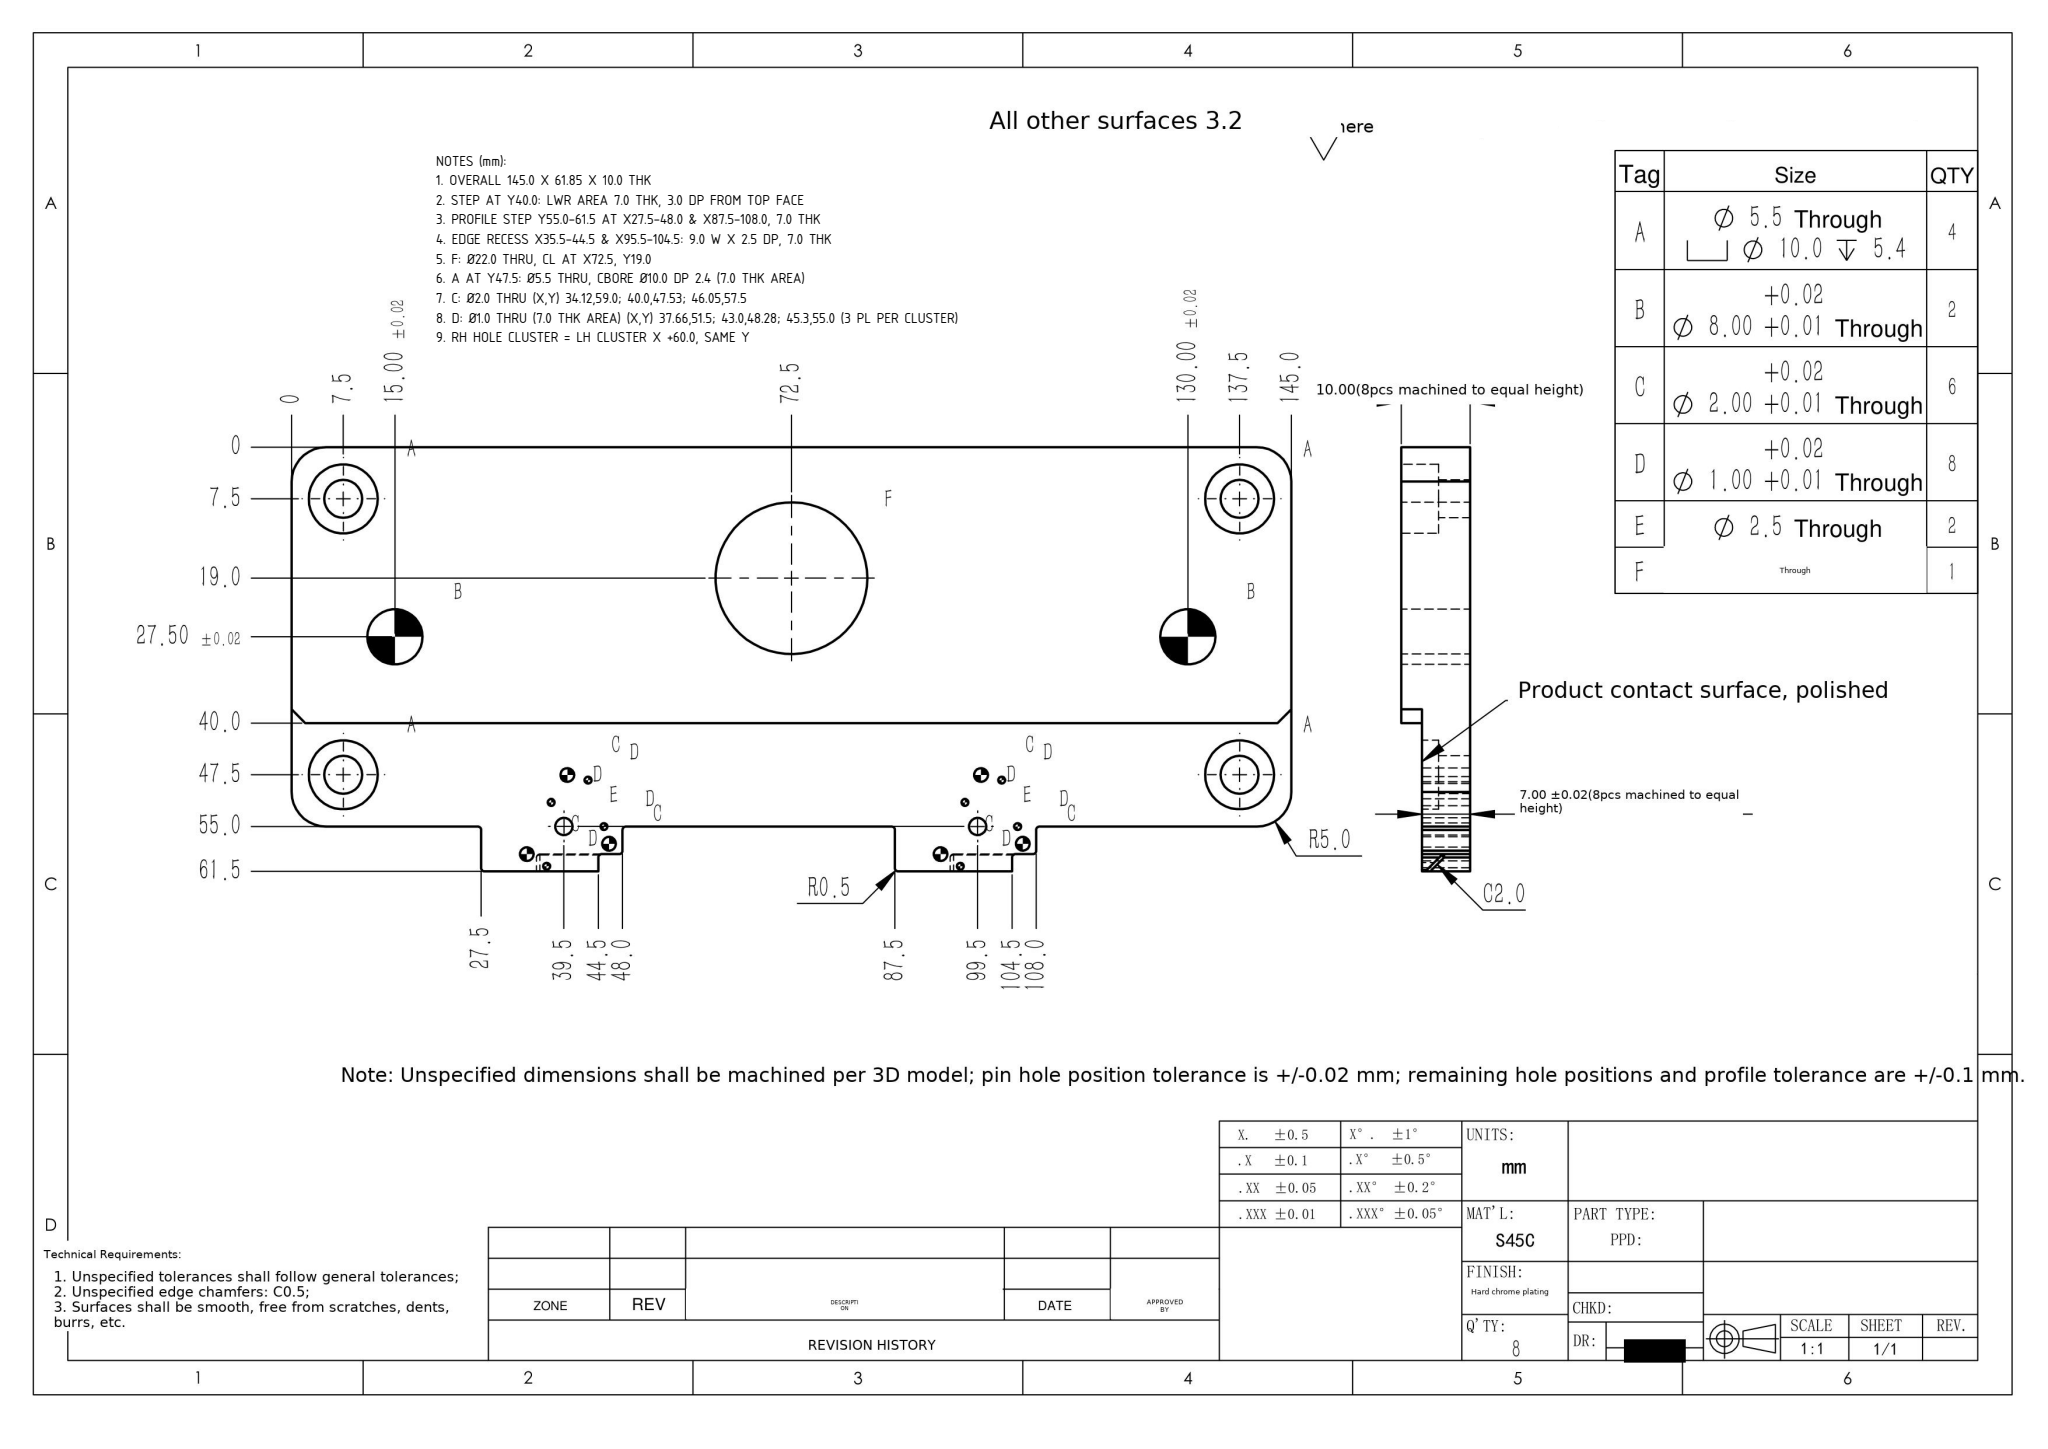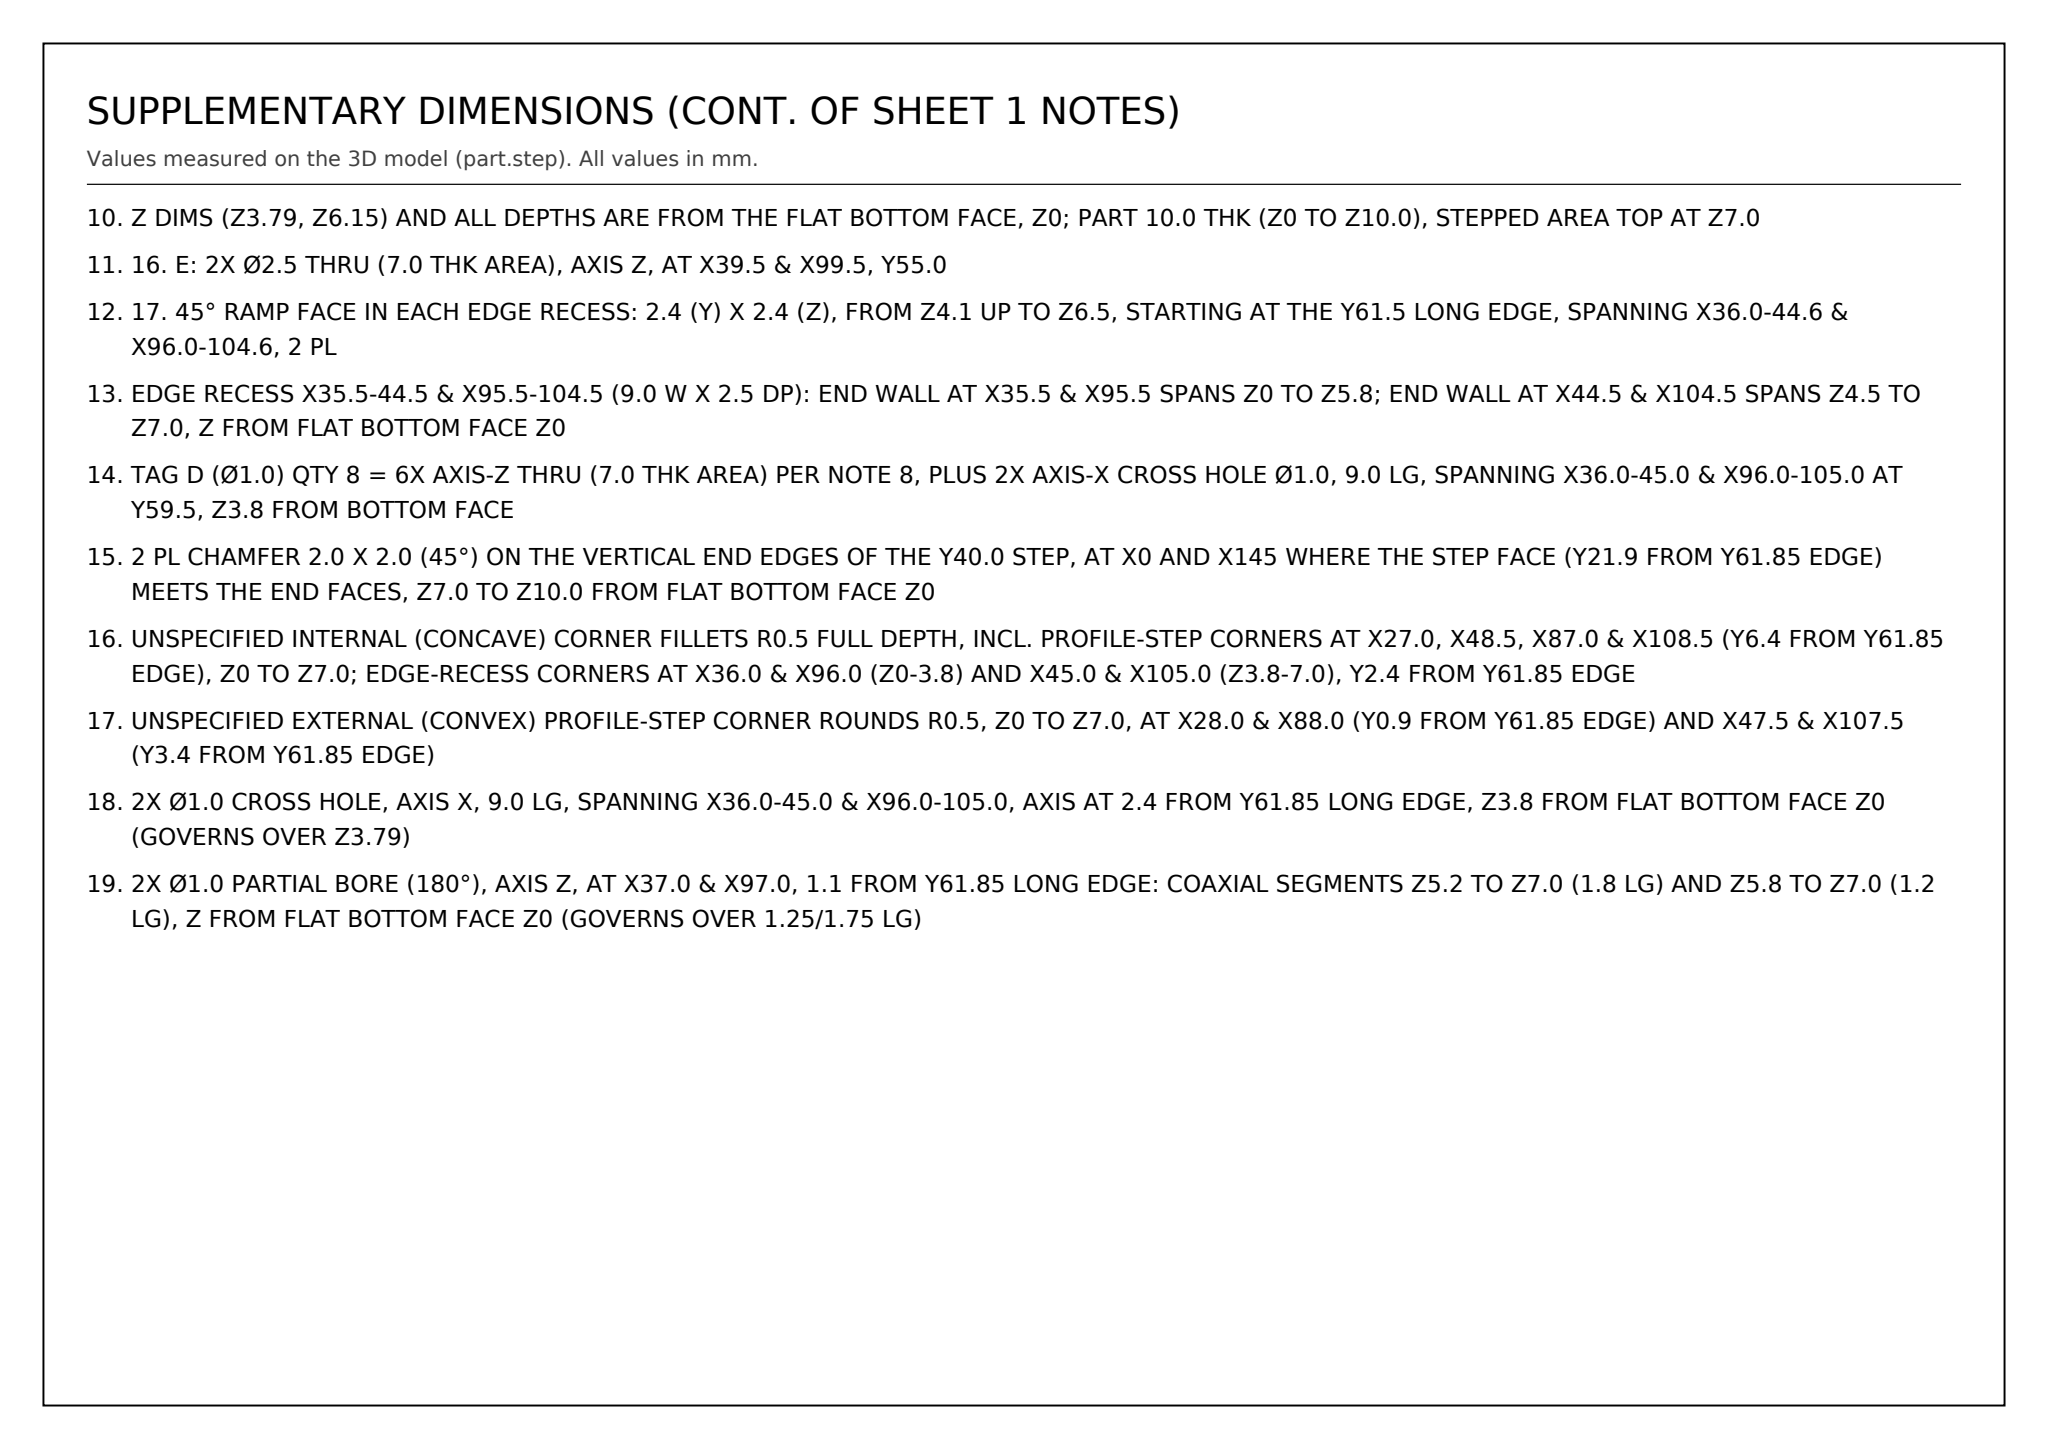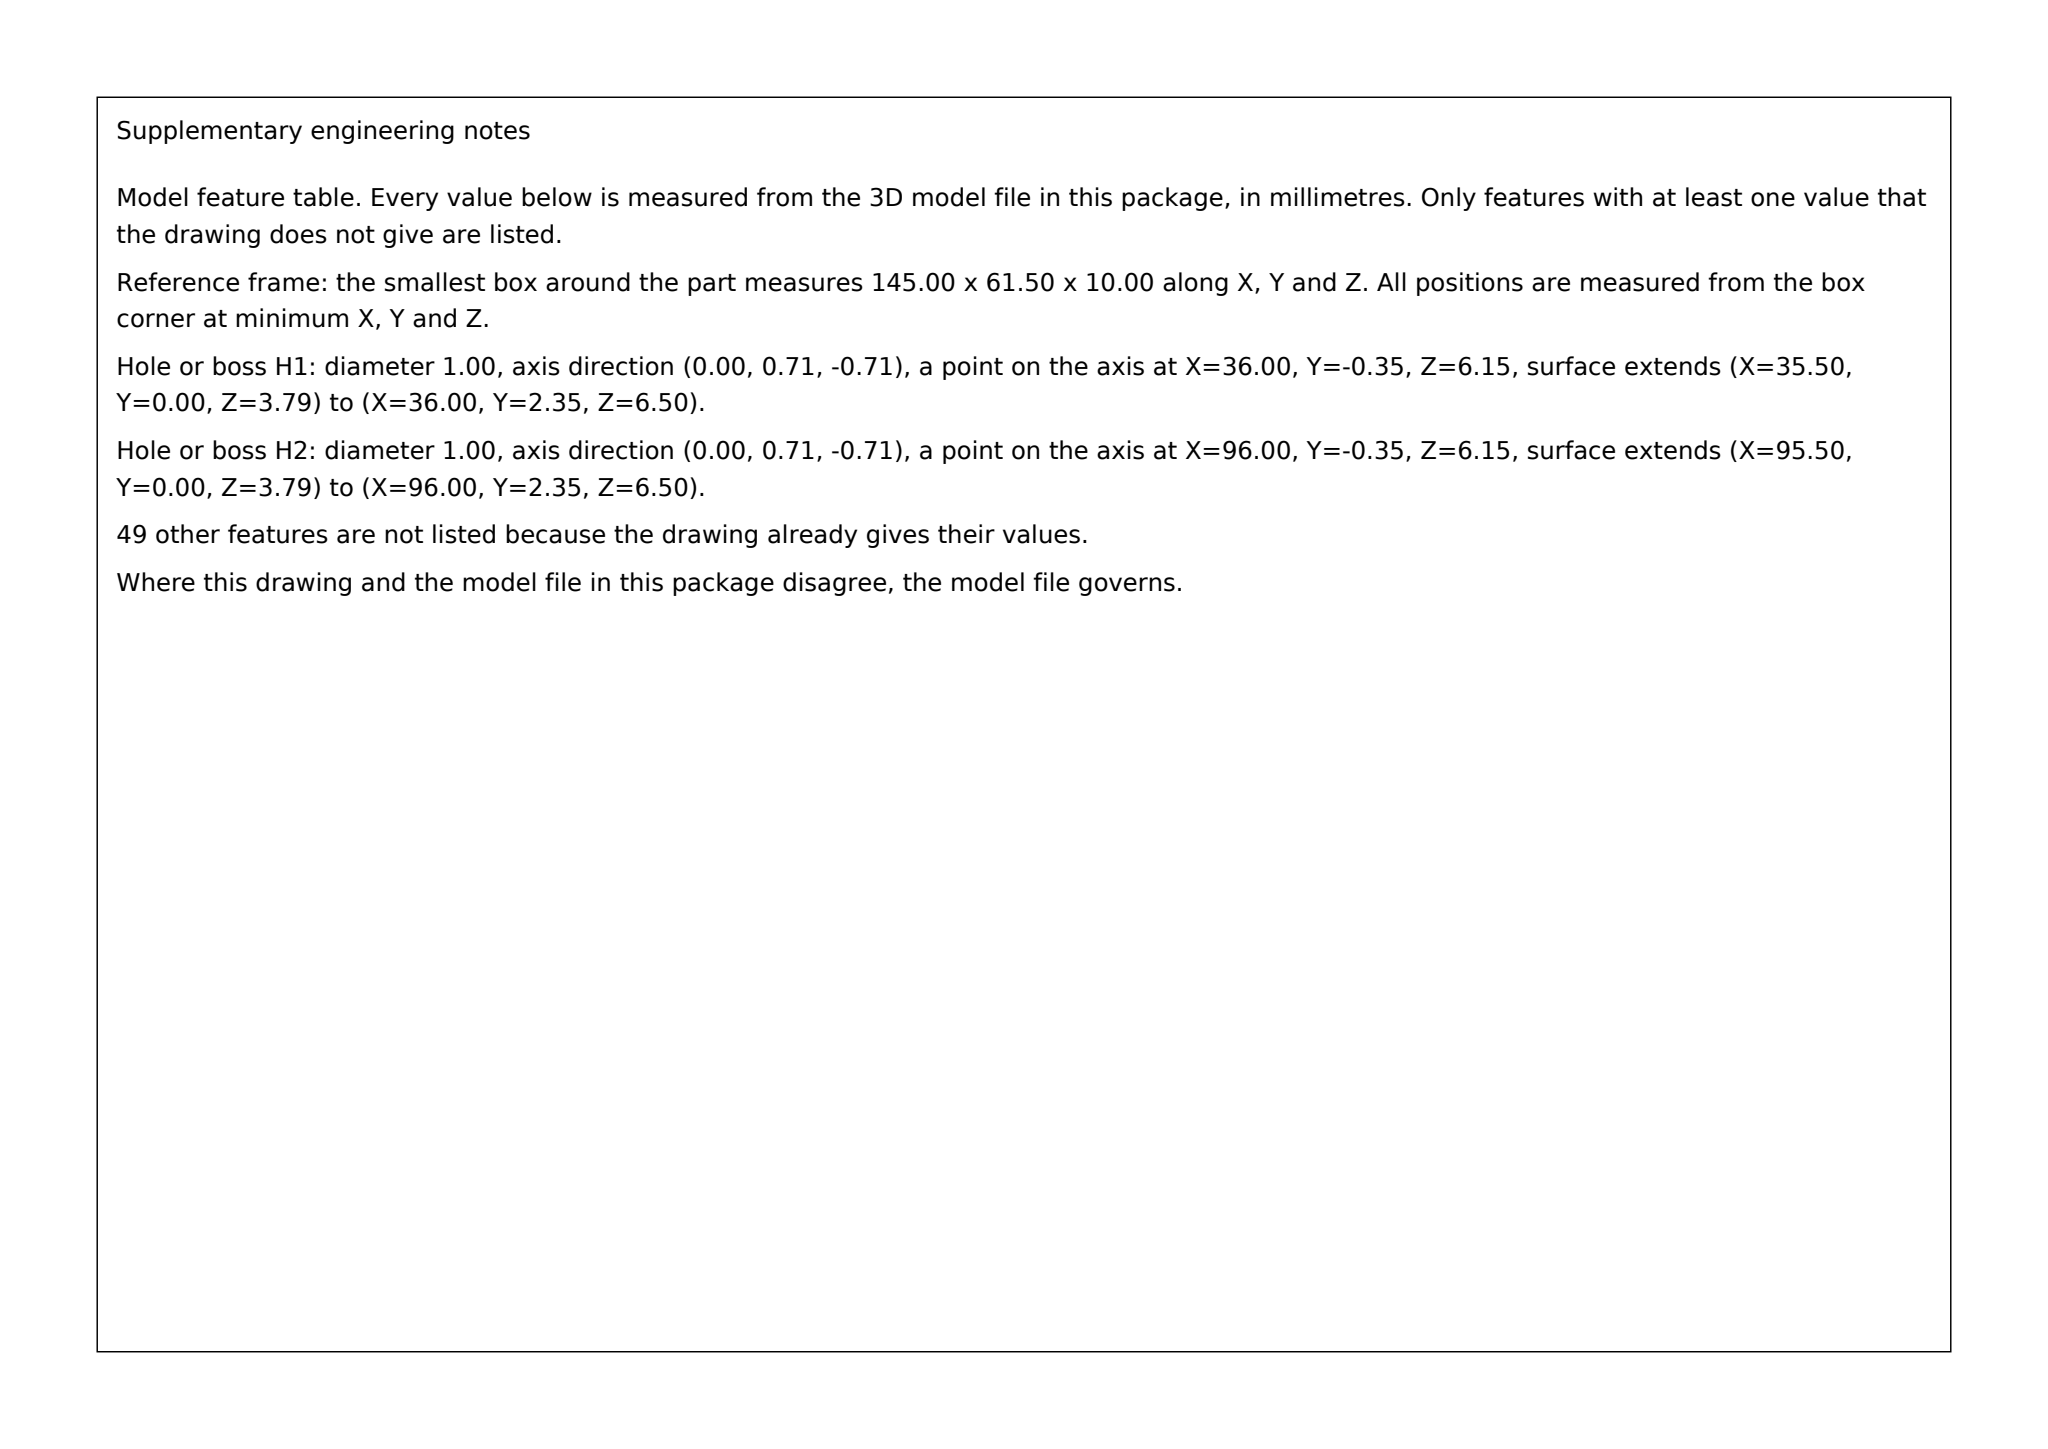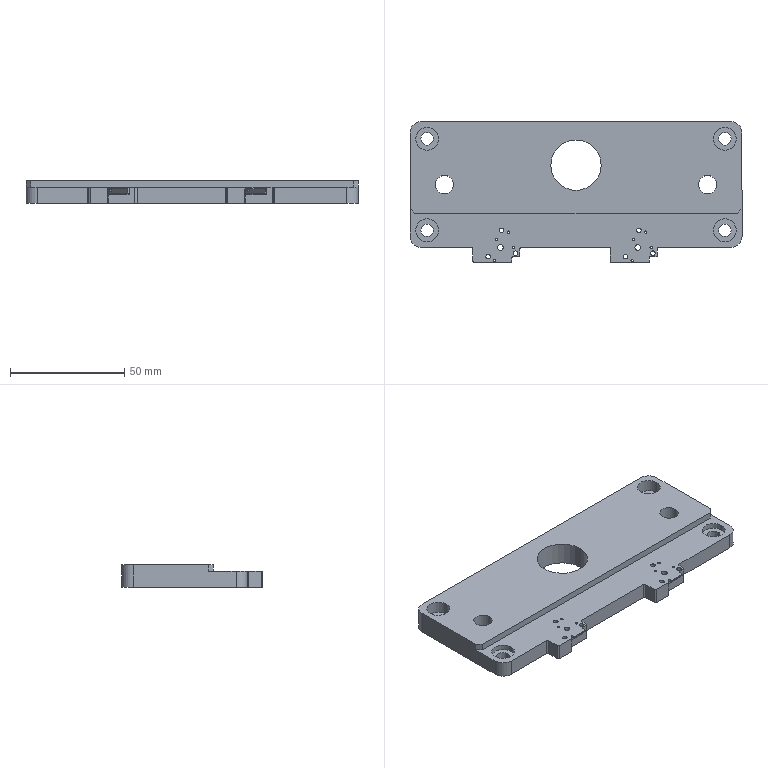Part | SolidWorks | mm | 1 solid | 106 faces | box 145 x 61.5 x 10 mm | volume 67834 mm3 | cylinder 74 | plane 30 | sphere 2 | commonest cylinder face diameters 1 x32 2 x12 10 x12 5.5 x8 2.5 x4 8 x4 22 x2
Drawing notes:
OVERALL 145.0 X 61.85 X 10.0 THK | from the solid: bbox_xyz [145.0, 61.854, 10.0]
STEP AT Y40.0: LWR AREA 7.0 THK, 3.0 DP FROM TOP FACE | from the solid: y plane 21.85 (=Y40.0); z planes 7.0 & 10.0; lower-area cyls len 7.0
PROFILE STEP Y55.0-61.5 AT X27.5-48.0 & X87.5-108.0, 7.0 THK | from the solid: x planes 27.5/48.0/87.5/108.0; y planes 6.85(=55.0) & 0.35(=61.5)
EDGE RECESS X35.5-44.5 & X95.5-104.5: 9.0 W X 2.5 DP, 7.0 THK | from the solid: x planes 35.5/44.5/95.5/104.5; y planes 2.85(=Y59.0) to 0.35(=Y61.5)
F: Ø22.0 THRU, CL AT X72.5, Y19.0 | from the solid: cyl dia 22.0 axis z at (72.5, 42.85) len 10.0; Y=61.854-42.85=19.0
A AT Y47.5: Ø5.5 THRU, CBORE Ø10.0 DP 2.4 (7.0 THK AREA) | from the solid: dia 10.0 z-cyls (7.5,14.35)&(137.5,14.35) len 2.4; dia 5.5 len 4.6
C: Ø2.0 THRU (X,Y) 34.12,59.0; 40.0,47.53; 46.05,57.5 | from the solid: dia 2.0 z-cyls (34.12,2.85)(40.0,14.32)(46.05,4.35) len 7.0; Y=61.854-y
D: Ø1.0 THRU (7.0 THK AREA) (X,Y) 37.66,51.5; 43.0,48.28; 45.3,55.0 (3 PL PER CLUSTER) | from the solid: Full 360° Ø1.0 z-axis holes running z0→z7 exist only at (37.7,10.4), (43.0,13.6), (45.3,6.9) and their +60.0 mirrors (97.7,10.4), (103.0,13.6), (105.3,6.9) = 6 total; drawing Y = 61.9 - y_step gives 51.5, 48.3, 55.0. The locations 27.0,55.5 / 28.0,61.0 / 47.5,58.5 / 48.5,55.5 are Ø1.0 90° concave/convex profile arcs (R0.5 corner fillets/rounds at x27.0,y6.4; x28.0,y0.9; x47.5,y3.4; x48.5,y6.4), not holes.
RH HOLE CLUSTER = LH CLUSTER X +60.0, SAME Y | from the solid: all cluster cyls repeat at x+60 (87/88/96/97/97.66/103/105.3/107.5/108.5)
Z DIMS (Z3.79, Z6.15) AND ALL DEPTHS ARE FROM THE FLAT BOTTOM FACE, Z0; PART 10.0 THK (Z0 TO Z10.0), STEPPED AREA TOP AT Z7.0 | from the solid: axis_planes z = 0.0, 7.0, 10.0; cross hole z=3.79; axis-Y hole z=6.15
16. E: 2X Ø2.5 THRU (7.0 THK AREA), AXIS Z, AT X39.5 & X99.5, Y55.0 | from the solid: cylinders: hole/bore Ø2.5 axis z at [39.5, 6.9] and [99.5, 6.9], from z0.0 to z7.0 (y 6.9 from min corner = Y55.0 from top datum, bbox_y 61.854)
17. 45° RAMP FACE IN EACH EDGE RECESS: 2.4 (Y) X 2.4 (Z), FROM Z4.1 UP TO Z6.5, STARTING AT THE Y61.5 LONG EDGE, SPANNING X36.0-44.6 & X96.0-104.6, 2 PL | from the solid: inclined_planes: angle_to_xyz_axes [90,45,45], bbox_from [36.0,0.4,4.1] and [96.0,0.4,4.1], size [8.6,2.4,2.4]
EDGE RECESS X35.5-44.5 & X95.5-104.5 (9.0 W X 2.5 DP): END WALL AT X35.5 & X95.5 SPANS Z0 TO Z5.8; END WALL AT X44.5 & X104.5 SPANS Z4.5 TO Z7.0, Z FROM FLAT BOTTOM FACE Z0 | from the solid: axis planes: x=35.5 extent z[0.0,5.8], x=95.5 extent z[0.0,5.8], x=44.5 extent z[4.5,7.0], x=104.5 extent z[4.5,7.0]
TAG D (Ø1.0) QTY 8 = 6X AXIS-Z THRU (7.0 THK AREA) PER NOTE 8, PLUS 2X AXIS-X CROSS HOLE Ø1.0, 9.0 LG, SPANNING X36.0-45.0 & X96.0-105.0 AT Y59.5, Z3.8 FROM BOTTOM FACE | from the solid: 6 full 360° dia 1.0 axis-z holes z0-7.0 at (37.7,10.4),(43.0,13.6),(45.3,6.9),(97.7,10.4),(103.0,13.6),(105.3,6.9); dia 1.0 axis-x cylinders at [y2.4,z3.8] from x36.0 to 45.0 and from x96.0 to 105.0
2 PL CHAMFER 2.0 X 2.0 (45°) ON THE VERTICAL END EDGES OF THE Y40.0 STEP, AT X0 AND X145 WHERE THE STEP FACE (Y21.9 FROM Y61.85 EDGE) MEETS THE END FACES, Z7.0 TO Z10.0 FROM FLAT BOTTOM FACE Z0 | from the solid: inclined_planes: angle_to_xyz_axes [45,45,90], bbox_from [0.0,21.9,7.0] and [143.0,21.9,7.0], size [2.0,2.0,3.0]
UNSPECIFIED INTERNAL (CONCAVE) CORNER FILLETS R0.5 FULL DEPTH, INCL. PROFILE-STEP CORNERS AT X27.0, X48.5, X87.0 & X108.5 (Y6.4 FROM Y61.85 EDGE), Z0 TO Z7.0; EDGE-RECESS CORNERS AT X36.0 & X96.0 (Z0-3.8) AND X45.0 & X105.0 (Z3.8-7.0), Y2.4 FROM Y61.85 EDGE | from the solid: cylinders: concave arc dia 1.0 axis z at [27.0,6.4],[48.5,6.4],[87.0,6.4],[108.5,6.4] from 0.0 to 7.0; concave arc dia 1.0 axis z at [36.0,2.4],[96.0,2.4] from 0.0 to 3.8 and [45.0,2.4],[105.0,2.4] from 3.8 to 7.0
UNSPECIFIED EXTERNAL (CONVEX) PROFILE-STEP CORNER ROUNDS R0.5, Z0 TO Z7.0, AT X28.0 & X88.0 (Y0.9 FROM Y61.85 EDGE) AND X47.5 & X107.5 (Y3.4 FROM Y61.85 EDGE) | from the solid: cylinders: convex arc dia 1.0 axis z at [28.0,0.9],[88.0,0.9],[47.5,3.4],[107.5,3.4], from 0.0 to 7.0
2X Ø1.0 CROSS HOLE, AXIS X, 9.0 LG, SPANNING X36.0-45.0 & X96.0-105.0, AXIS AT 2.4 FROM Y61.85 LONG EDGE, Z3.8 FROM FLAT BOTTOM FACE Z0 (GOVERNS OVER Z3.79) | from the solid: cylinders: concave arc dia 1.0 axis x, axis_pos [y 2.4, z 3.8], from 36.0 to 45.0 and from 96.0 to 105.0
2X Ø1.0 PARTIAL BORE (180°), AXIS Z, AT X37.0 & X97.0, 1.1 FROM Y61.85 LONG EDGE: COAXIAL SEGMENTS Z5.2 TO Z7.0 (1.8 LG) AND Z5.8 TO Z7.0 (1.2 LG), Z FROM FLAT BOTTOM FACE Z0 (GOVERNS OVER 1.25/1.75 LG) | from the solid: cylinders: concave arc dia 1.0 axis z at [37.0,1.1] and [97.0,1.1], from 5.2 to 7.0 and from 5.8 to 7.0, arc_deg 180